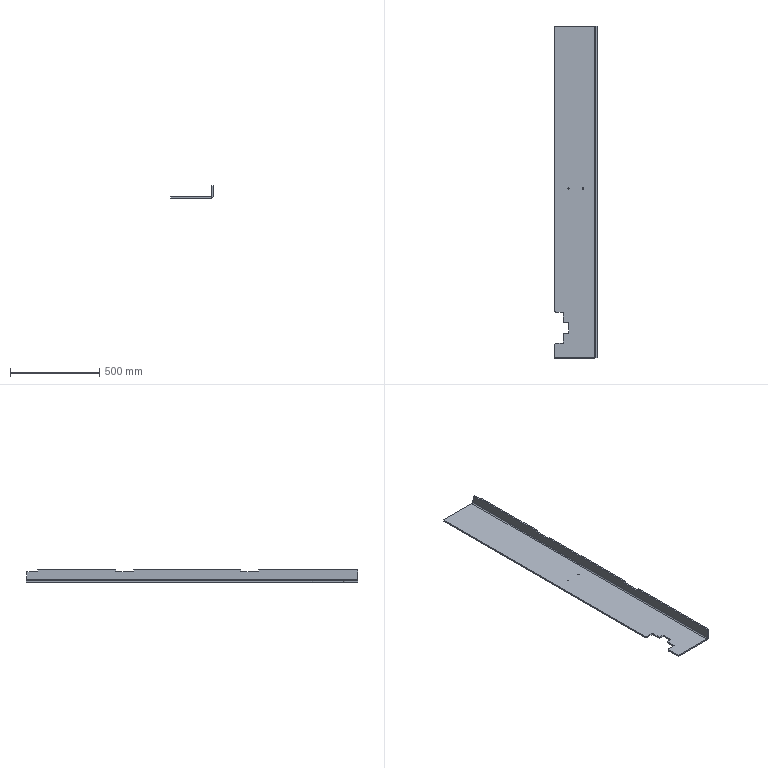Component | SolidWorks | BoxSupport,Left-1 | 1 solid | 41 faces | volume 4277935 mm3 | plane 33 | cylinder 8 | commonest cylinder face diameters 6.8 x4 20 x2 12 x1 28 x1 | material Q235